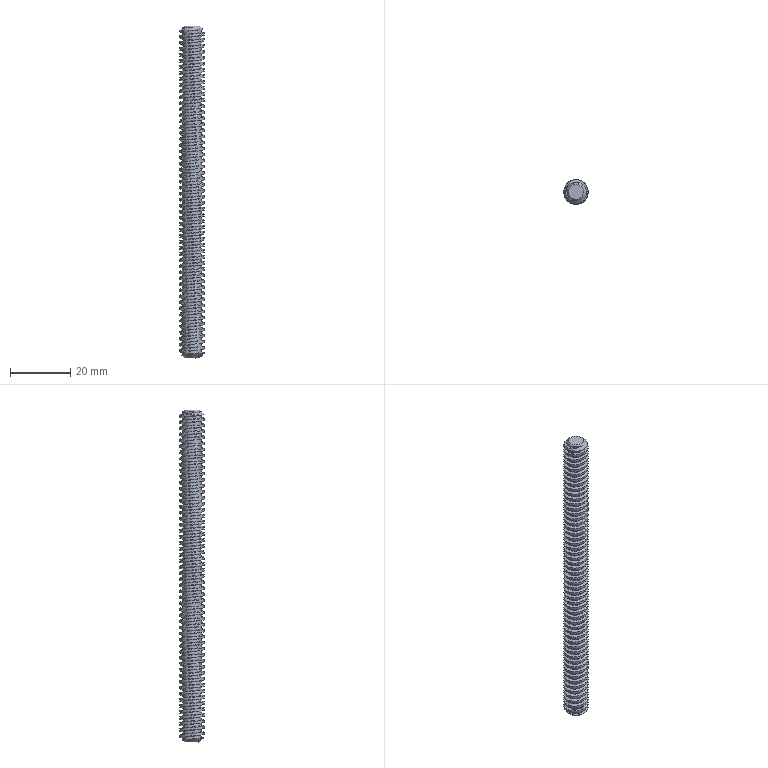Component | NX | LEADSCREW | 1 solid | 10 faces | volume 4275 mm3 | plane 3 | cone 3 | cylinder 2 | spline 2 | commonest cylinder face diameters 8 x1 6 x1